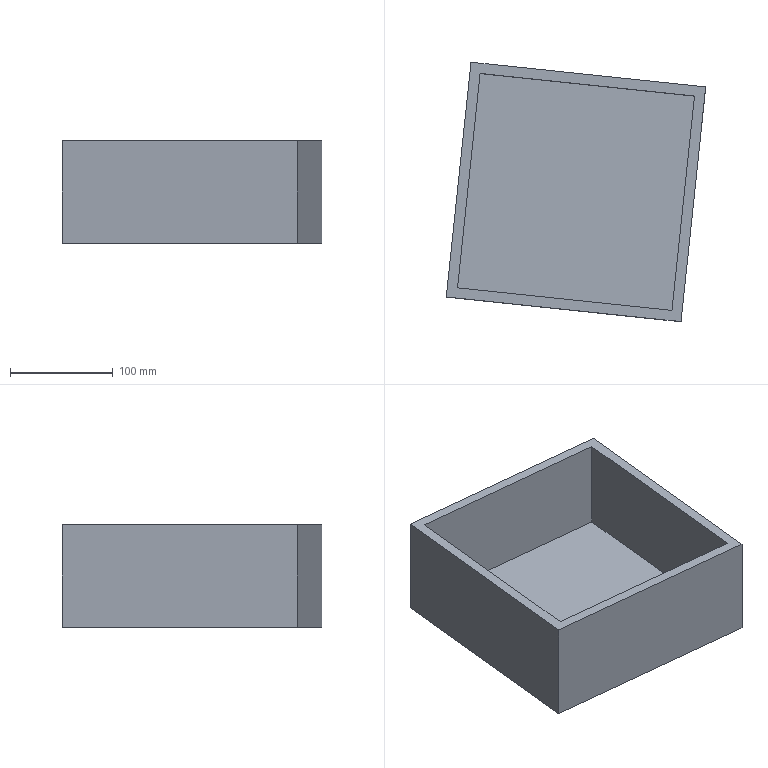Component | NX | SQUARE_BOX | 1 solid | 11 faces | box 252.78 x 252.78 x 100 mm | volume 1321000 mm3 | plane 11
STEP:
#1=CARTESIAN_POINT('',(0.,0.,0.));
#2=DIRECTION('',(0.,0.,1.));
#3=DIRECTION('',(1.,0.,0.));
#4=AXIS2_PLACEMENT_3D('',#1,#2,#3);
#5=CARTESIAN_POINT('',(-42.53,33.666,104.));
#6=VERTEX_POINT('',#5);
#7=CARTESIAN_POINT('',(-66.572,-195.074,104.));
#8=VERTEX_POINT('',#7);
#9=CARTESIAN_POINT('',(-54.551,-80.704,104.));
#10=DIRECTION('',(-0.1045,-0.9945,0.));
#11=VECTOR('',#10,1.);
#12=LINE('',#9,#11);
#13=CARTESIAN_POINT('',(-168.921,-68.683,104.));
#14=DIRECTION('',(0.,0.,1.));
#15=DIRECTION('',(0.1045,0.9945,0.));
#16=AXIS2_PLACEMENT_3D('',#13,#14,#15);
#17=PLANE('',#16);
#18=CARTESIAN_POINT('',(0.,-115.));
#19=DIRECTION('',(-1.,0.));
#20=VECTOR('',#19,1.);
#21=LINE('',#18,#20);
#22=(GEOMETRIC_REPRESENTATION_CONTEXT(2)PARAMETRIC_REPRESENTATION_CONTEXT()REPRESENTATION_CONTEXT('',''));
#23=DEFINITIONAL_REPRESENTATION('',(#21),#22);
#24=PCURVE('',#17,#23);
#25=CARTESIAN_POINT('',(-54.551,-80.704,4.));
#26=DIRECTION('',(0.9945,-0.1045,0.));
#27=DIRECTION('',(0.,0.,-1.));
#28=AXIS2_PLACEMENT_3D('',#25,#26,#27);
#29=PLANE('',#28);
#30=CARTESIAN_POINT('',(-100.,0.));
#31=DIRECTION('',(0.,-1.));
#32=VECTOR('',#31,1.);
#33=LINE('',#30,#32);
#34=(GEOMETRIC_REPRESENTATION_CONTEXT(2)PARAMETRIC_REPRESENTATION_CONTEXT()REPRESENTATION_CONTEXT('',''));
#35=DEFINITIONAL_REPRESENTATION('',(#33),#34);
#36=PCURVE('',#29,#35);
#37=SURFACE_CURVE('',#12,(#24,#36),.PCURVE_S1.);
#38=EDGE_CURVE('',#6,#8,#37,.T.);
#39=ORIENTED_EDGE('',*,*,#38,.F.);
#40=CARTESIAN_POINT('',(-271.27,57.707,104.));
#41=VERTEX_POINT('',#40);
#42=CARTESIAN_POINT('',(-156.9,45.687,104.));
#43=DIRECTION('',(0.9945,-0.1045,0.));
#44=VECTOR('',#43,1.);
#45=LINE('',#42,#44);
#46=CARTESIAN_POINT('',(115.,0.));
#47=DIRECTION('',(0.,-1.));
#48=VECTOR('',#47,1.);
#49=LINE('',#46,#48);
#50=(GEOMETRIC_REPRESENTATION_CONTEXT(2)PARAMETRIC_REPRESENTATION_CONTEXT()REPRESENTATION_CONTEXT('',''));
#51=DEFINITIONAL_REPRESENTATION('',(#49),#50);
#52=PCURVE('',#17,#51);
#53=CARTESIAN_POINT('',(-156.9,45.687,4.));
#54=DIRECTION('',(0.1045,0.9945,0.));
#55=DIRECTION('',(0.,0.,-1.));
#56=AXIS2_PLACEMENT_3D('',#53,#54,#55);
#57=PLANE('',#56);
#58=CARTESIAN_POINT('',(-100.,0.));
#59=DIRECTION('',(0.,-1.));
#60=VECTOR('',#59,1.);
#61=LINE('',#58,#60);
#62=(GEOMETRIC_REPRESENTATION_CONTEXT(2)PARAMETRIC_REPRESENTATION_CONTEXT()REPRESENTATION_CONTEXT('',''));
#63=DEFINITIONAL_REPRESENTATION('',(#61),#62);
#64=PCURVE('',#57,#63);
#65=SURFACE_CURVE('',#45,(#52,#64),.PCURVE_S1.);
#66=EDGE_CURVE('',#41,#6,#65,.T.);
#67=ORIENTED_EDGE('',*,*,#66,.F.);
#68=CARTESIAN_POINT('',(-295.312,-171.033,104.));
#69=VERTEX_POINT('',#68);
#70=CARTESIAN_POINT('',(-283.291,-56.663,104.));
#71=DIRECTION('',(0.1045,0.9945,0.));
#72=VECTOR('',#71,1.);
#73=LINE('',#70,#72);
#74=CARTESIAN_POINT('',(0.,115.));
#75=DIRECTION('',(1.,0.));
#76=VECTOR('',#75,1.);
#77=LINE('',#74,#76);
#78=(GEOMETRIC_REPRESENTATION_CONTEXT(2)PARAMETRIC_REPRESENTATION_CONTEXT()REPRESENTATION_CONTEXT('',''));
#79=DEFINITIONAL_REPRESENTATION('',(#77),#78);
#80=PCURVE('',#17,#79);
#81=CARTESIAN_POINT('',(-283.291,-56.663,4.));
#82=DIRECTION('',(-0.9945,0.1045,0.));
#83=DIRECTION('',(0.,0.,1.));
#84=AXIS2_PLACEMENT_3D('',#81,#82,#83);
#85=PLANE('',#84);
#86=CARTESIAN_POINT('',(100.,0.));
#87=DIRECTION('',(0.,1.));
#88=VECTOR('',#87,1.);
#89=LINE('',#86,#88);
#90=(GEOMETRIC_REPRESENTATION_CONTEXT(2)PARAMETRIC_REPRESENTATION_CONTEXT()REPRESENTATION_CONTEXT('',''));
#91=DEFINITIONAL_REPRESENTATION('',(#89),#90);
#92=PCURVE('',#85,#91);
#93=SURFACE_CURVE('',#73,(#80,#92),.PCURVE_S1.);
#94=EDGE_CURVE('',#69,#41,#93,.T.);
#95=ORIENTED_EDGE('',*,*,#94,.F.);
#96=CARTESIAN_POINT('',(-180.942,-183.053,104.));
#97=DIRECTION('',(-0.9945,0.1045,0.));
#98=VECTOR('',#97,1.);
#99=LINE('',#96,#98);
#100=CARTESIAN_POINT('',(-115.,-0.));
#101=DIRECTION('',(0.,1.));
#102=VECTOR('',#101,1.);
#103=LINE('',#100,#102);
#104=(GEOMETRIC_REPRESENTATION_CONTEXT(2)PARAMETRIC_REPRESENTATION_CONTEXT()REPRESENTATION_CONTEXT('',''));
#105=DEFINITIONAL_REPRESENTATION('',(#103),#104);
#106=PCURVE('',#17,#105);
#107=CARTESIAN_POINT('',(-180.942,-183.053,4.));
#108=DIRECTION('',(-0.1045,-0.9945,0.));
#109=DIRECTION('',(0.,0.,1.));
#110=AXIS2_PLACEMENT_3D('',#107,#108,#109);
#111=PLANE('',#110);
#112=CARTESIAN_POINT('',(100.,0.));
#113=DIRECTION('',(0.,1.));
#114=VECTOR('',#113,1.);
#115=LINE('',#112,#114);
#116=(GEOMETRIC_REPRESENTATION_CONTEXT(2)PARAMETRIC_REPRESENTATION_CONTEXT()REPRESENTATION_CONTEXT('',''));
#117=DEFINITIONAL_REPRESENTATION('',(#115),#116);
#118=PCURVE('',#111,#117);
#119=SURFACE_CURVE('',#99,(#106,#118),.PCURVE_S1.);
#120=EDGE_CURVE('',#8,#69,#119,.T.);
#121=ORIENTED_EDGE('',*,*,#120,.F.);
#122=EDGE_LOOP('',(#39,#67,#95,#121));
#123=FACE_BOUND('',#122,.T.);
#124=CARTESIAN_POINT('',(-262.37,46.717,104.));
#125=VERTEX_POINT('',#124);
#126=CARTESIAN_POINT('',(-53.521,24.766,104.));
#127=VERTEX_POINT('',#126);
#128=CARTESIAN_POINT('',(-157.946,35.741,104.));
#129=DIRECTION('',(0.9945,-0.1045,0.));
#130=VECTOR('',#129,1.);
#131=LINE('',#128,#130);
#132=CARTESIAN_POINT('',(105.,-0.));
#133=DIRECTION('',(0.,-1.));
#134=VECTOR('',#133,1.);
#135=LINE('',#132,#134);
#136=(GEOMETRIC_REPRESENTATION_CONTEXT(2)PARAMETRIC_REPRESENTATION_CONTEXT()REPRESENTATION_CONTEXT('',''));
#137=DEFINITIONAL_REPRESENTATION('',(#135),#136);
#138=PCURVE('',#17,#137);
#139=CARTESIAN_POINT('',(-157.946,35.741,4.));
#140=DIRECTION('',(0.1045,0.9945,0.));
#141=DIRECTION('',(0.,0.,-1.));
#142=AXIS2_PLACEMENT_3D('',#139,#140,#141);
#143=PLANE('',#142);
#144=CARTESIAN_POINT('',(-100.,0.));
#145=DIRECTION('',(0.,-1.));
#146=VECTOR('',#145,1.);
#147=LINE('',#144,#146);
#148=(GEOMETRIC_REPRESENTATION_CONTEXT(2)PARAMETRIC_REPRESENTATION_CONTEXT()REPRESENTATION_CONTEXT('',''));
#149=DEFINITIONAL_REPRESENTATION('',(#147),#148);
#150=PCURVE('',#143,#149);
#151=SURFACE_CURVE('',#131,(#138,#150),.PCURVE_S1.);
#152=EDGE_CURVE('',#125,#127,#151,.T.);
#153=ORIENTED_EDGE('',*,*,#152,.T.);
#154=CARTESIAN_POINT('',(-75.472,-184.084,104.));
#155=VERTEX_POINT('',#154);
#156=CARTESIAN_POINT('',(-64.496,-79.659,104.));
#157=DIRECTION('',(-0.1045,-0.9945,0.));
#158=VECTOR('',#157,1.);
#159=LINE('',#156,#158);
#160=CARTESIAN_POINT('',(-0.,-105.));
#161=DIRECTION('',(-1.,0.));
#162=VECTOR('',#161,1.);
#163=LINE('',#160,#162);
#164=(GEOMETRIC_REPRESENTATION_CONTEXT(2)PARAMETRIC_REPRESENTATION_CONTEXT()REPRESENTATION_CONTEXT('',''));
#165=DEFINITIONAL_REPRESENTATION('',(#163),#164);
#166=PCURVE('',#17,#165);
#167=CARTESIAN_POINT('',(-64.496,-79.659,4.));
#168=DIRECTION('',(0.9945,-0.1045,0.));
#169=DIRECTION('',(0.,0.,-1.));
#170=AXIS2_PLACEMENT_3D('',#167,#168,#169);
#171=PLANE('',#170);
#172=CARTESIAN_POINT('',(-100.,0.));
#173=DIRECTION('',(0.,-1.));
#174=VECTOR('',#173,1.);
#175=LINE('',#172,#174);
#176=(GEOMETRIC_REPRESENTATION_CONTEXT(2)PARAMETRIC_REPRESENTATION_CONTEXT()REPRESENTATION_CONTEXT('',''));
#177=DEFINITIONAL_REPRESENTATION('',(#175),#176);
#178=PCURVE('',#171,#177);
#179=SURFACE_CURVE('',#159,(#166,#178),.PCURVE_S1.);
#180=EDGE_CURVE('',#127,#155,#179,.T.);
#181=ORIENTED_EDGE('',*,*,#180,.T.);
#182=CARTESIAN_POINT('',(-284.321,-162.133,104.));
#183=VERTEX_POINT('',#182);
#184=CARTESIAN_POINT('',(-179.897,-173.108,104.));
#185=DIRECTION('',(-0.9945,0.1045,0.));
#186=VECTOR('',#185,1.);
#187=LINE('',#184,#186);
#188=CARTESIAN_POINT('',(-105.,-0.));
#189=DIRECTION('',(0.,1.));
#190=VECTOR('',#189,1.);
#191=LINE('',#188,#190);
#192=(GEOMETRIC_REPRESENTATION_CONTEXT(2)PARAMETRIC_REPRESENTATION_CONTEXT()REPRESENTATION_CONTEXT('',''));
#193=DEFINITIONAL_REPRESENTATION('',(#191),#192);
#194=PCURVE('',#17,#193);
#195=CARTESIAN_POINT('',(-179.897,-173.108,4.));
#196=DIRECTION('',(-0.1045,-0.9945,0.));
#197=DIRECTION('',(0.,0.,1.));
#198=AXIS2_PLACEMENT_3D('',#195,#196,#197);
#199=PLANE('',#198);
#200=CARTESIAN_POINT('',(100.,0.));
#201=DIRECTION('',(0.,1.));
#202=VECTOR('',#201,1.);
#203=LINE('',#200,#202);
#204=(GEOMETRIC_REPRESENTATION_CONTEXT(2)PARAMETRIC_REPRESENTATION_CONTEXT()REPRESENTATION_CONTEXT('',''));
#205=DEFINITIONAL_REPRESENTATION('',(#203),#204);
#206=PCURVE('',#199,#205);
#207=SURFACE_CURVE('',#187,(#194,#206),.PCURVE_S1.);
#208=EDGE_CURVE('',#155,#183,#207,.T.);
#209=ORIENTED_EDGE('',*,*,#208,.T.);
#210=CARTESIAN_POINT('',(-273.346,-57.708,104.));
#211=DIRECTION('',(0.1045,0.9945,0.));
#212=VECTOR('',#211,1.);
#213=LINE('',#210,#212);
#214=CARTESIAN_POINT('',(0.,105.));
#215=DIRECTION('',(1.,0.));
#216=VECTOR('',#215,1.);
#217=LINE('',#214,#216);
#218=(GEOMETRIC_REPRESENTATION_CONTEXT(2)PARAMETRIC_REPRESENTATION_CONTEXT()REPRESENTATION_CONTEXT('',''));
#219=DEFINITIONAL_REPRESENTATION('',(#217),#218);
#220=PCURVE('',#17,#219);
#221=CARTESIAN_POINT('',(-273.346,-57.708,4.));
#222=DIRECTION('',(-0.9945,0.1045,0.));
#223=DIRECTION('',(0.,0.,1.));
#224=AXIS2_PLACEMENT_3D('',#221,#222,#223);
#225=PLANE('',#224);
#226=CARTESIAN_POINT('',(100.,0.));
#227=DIRECTION('',(0.,1.));
#228=VECTOR('',#227,1.);
#229=LINE('',#226,#228);
#230=(GEOMETRIC_REPRESENTATION_CONTEXT(2)PARAMETRIC_REPRESENTATION_CONTEXT()REPRESENTATION_CONTEXT('',''));
#231=DEFINITIONAL_REPRESENTATION('',(#229),#230);
#232=PCURVE('',#225,#231);
#233=SURFACE_CURVE('',#213,(#220,#232),.PCURVE_S1.);
#234=EDGE_CURVE('',#183,#125,#233,.T.);
#235=ORIENTED_EDGE('',*,*,#234,.T.);
#236=EDGE_LOOP('',(#153,#181,#209,#235));
#237=FACE_BOUND('',#236,.T.);
#238=ADVANCED_FACE('',(#123,#237),#17,.T.);
#239=CARTESIAN_POINT('',(-42.53,33.666,4.));
#240=VERTEX_POINT('',#239);
#241=CARTESIAN_POINT('',(-42.53,33.666,4.));
#242=DIRECTION('',(0.,0.,1.));
#243=VECTOR('',#242,1.);
#244=LINE('',#241,#243);
#245=CARTESIAN_POINT('',(0.,115.));
#246=DIRECTION('',(-1.,0.));
#247=VECTOR('',#246,1.);
#248=LINE('',#245,#247);
#249=(GEOMETRIC_REPRESENTATION_CONTEXT(2)PARAMETRIC_REPRESENTATION_CONTEXT()REPRESENTATION_CONTEXT('',''));
#250=DEFINITIONAL_REPRESENTATION('',(#248),#249);
#251=PCURVE('',#29,#250);
#252=CARTESIAN_POINT('',(0.,-115.));
#253=DIRECTION('',(-1.,0.));
#254=VECTOR('',#253,1.);
#255=LINE('',#252,#254);
#256=(GEOMETRIC_REPRESENTATION_CONTEXT(2)PARAMETRIC_REPRESENTATION_CONTEXT()REPRESENTATION_CONTEXT('',''));
#257=DEFINITIONAL_REPRESENTATION('',(#255),#256);
#258=PCURVE('',#57,#257);
#259=SURFACE_CURVE('',#244,(#251,#258),.PCURVE_S1.);
#260=EDGE_CURVE('',#240,#6,#259,.T.);
#261=ORIENTED_EDGE('',*,*,#260,.T.);
#262=ORIENTED_EDGE('',*,*,#38,.T.);
#263=CARTESIAN_POINT('',(-66.572,-195.074,4.));
#264=VERTEX_POINT('',#263);
#265=CARTESIAN_POINT('',(-66.572,-195.074,4.));
#266=DIRECTION('',(0.,0.,1.));
#267=VECTOR('',#266,1.);
#268=LINE('',#265,#267);
#269=CARTESIAN_POINT('',(0.,-115.));
#270=DIRECTION('',(-1.,0.));
#271=VECTOR('',#270,1.);
#272=LINE('',#269,#271);
#273=(GEOMETRIC_REPRESENTATION_CONTEXT(2)PARAMETRIC_REPRESENTATION_CONTEXT()REPRESENTATION_CONTEXT('',''));
#274=DEFINITIONAL_REPRESENTATION('',(#272),#273);
#275=PCURVE('',#29,#274);
#276=CARTESIAN_POINT('',(0.,-115.));
#277=DIRECTION('',(1.,0.));
#278=VECTOR('',#277,1.);
#279=LINE('',#276,#278);
#280=(GEOMETRIC_REPRESENTATION_CONTEXT(2)PARAMETRIC_REPRESENTATION_CONTEXT()REPRESENTATION_CONTEXT('',''));
#281=DEFINITIONAL_REPRESENTATION('',(#279),#280);
#282=PCURVE('',#111,#281);
#283=SURFACE_CURVE('',#268,(#275,#282),.PCURVE_S1.);
#284=EDGE_CURVE('',#264,#8,#283,.T.);
#285=ORIENTED_EDGE('',*,*,#284,.F.);
#286=CARTESIAN_POINT('',(-54.551,-80.704,4.));
#287=DIRECTION('',(0.1045,0.9945,0.));
#288=VECTOR('',#287,1.);
#289=LINE('',#286,#288);
#290=CARTESIAN_POINT('',(0.,0.));
#291=DIRECTION('',(0.,1.));
#292=VECTOR('',#291,1.);
#293=LINE('',#290,#292);
#294=(GEOMETRIC_REPRESENTATION_CONTEXT(2)PARAMETRIC_REPRESENTATION_CONTEXT()REPRESENTATION_CONTEXT('',''));
#295=DEFINITIONAL_REPRESENTATION('',(#293),#294);
#296=PCURVE('',#29,#295);
#297=CARTESIAN_POINT('',(-168.921,-68.683,4.));
#298=DIRECTION('',(0.,0.,-1.));
#299=DIRECTION('',(-0.1045,-0.9945,0.));
#300=AXIS2_PLACEMENT_3D('',#297,#298,#299);
#301=PLANE('',#300);
#302=CARTESIAN_POINT('',(-0.,-115.));
#303=DIRECTION('',(-1.,0.));
#304=VECTOR('',#303,1.);
#305=LINE('',#302,#304);
#306=(GEOMETRIC_REPRESENTATION_CONTEXT(2)PARAMETRIC_REPRESENTATION_CONTEXT()REPRESENTATION_CONTEXT('',''));
#307=DEFINITIONAL_REPRESENTATION('',(#305),#306);
#308=PCURVE('',#301,#307);
#309=SURFACE_CURVE('',#289,(#296,#308),.PCURVE_S1.);
#310=EDGE_CURVE('',#264,#240,#309,.T.);
#311=ORIENTED_EDGE('',*,*,#310,.T.);
#312=EDGE_LOOP('',(#261,#262,#285,#311));
#313=FACE_BOUND('',#312,.T.);
#314=ADVANCED_FACE('',(#313),#29,.T.);
#315=ORIENTED_EDGE('',*,*,#284,.T.);
#316=ORIENTED_EDGE('',*,*,#120,.T.);
#317=CARTESIAN_POINT('',(-295.312,-171.033,4.));
#318=VERTEX_POINT('',#317);
#319=CARTESIAN_POINT('',(-295.312,-171.033,4.));
#320=DIRECTION('',(0.,0.,1.));
#321=VECTOR('',#320,1.);
#322=LINE('',#319,#321);
#323=CARTESIAN_POINT('',(0.,115.));
#324=DIRECTION('',(1.,0.));
#325=VECTOR('',#324,1.);
#326=LINE('',#323,#325);
#327=(GEOMETRIC_REPRESENTATION_CONTEXT(2)PARAMETRIC_REPRESENTATION_CONTEXT()REPRESENTATION_CONTEXT('',''));
#328=DEFINITIONAL_REPRESENTATION('',(#326),#327);
#329=PCURVE('',#111,#328);
#330=CARTESIAN_POINT('',(0.,-115.));
#331=DIRECTION('',(1.,0.));
#332=VECTOR('',#331,1.);
#333=LINE('',#330,#332);
#334=(GEOMETRIC_REPRESENTATION_CONTEXT(2)PARAMETRIC_REPRESENTATION_CONTEXT()REPRESENTATION_CONTEXT('',''));
#335=DEFINITIONAL_REPRESENTATION('',(#333),#334);
#336=PCURVE('',#85,#335);
#337=SURFACE_CURVE('',#322,(#329,#336),.PCURVE_S1.);
#338=EDGE_CURVE('',#318,#69,#337,.T.);
#339=ORIENTED_EDGE('',*,*,#338,.F.);
#340=CARTESIAN_POINT('',(-180.942,-183.053,4.));
#341=DIRECTION('',(0.9945,-0.1045,0.));
#342=VECTOR('',#341,1.);
#343=LINE('',#340,#342);
#344=CARTESIAN_POINT('',(0.,0.));
#345=DIRECTION('',(0.,-1.));
#346=VECTOR('',#345,1.);
#347=LINE('',#344,#346);
#348=(GEOMETRIC_REPRESENTATION_CONTEXT(2)PARAMETRIC_REPRESENTATION_CONTEXT()REPRESENTATION_CONTEXT('',''));
#349=DEFINITIONAL_REPRESENTATION('',(#347),#348);
#350=PCURVE('',#111,#349);
#351=CARTESIAN_POINT('',(115.,-0.));
#352=DIRECTION('',(-0.,-1.));
#353=VECTOR('',#352,1.);
#354=LINE('',#351,#353);
#355=(GEOMETRIC_REPRESENTATION_CONTEXT(2)PARAMETRIC_REPRESENTATION_CONTEXT()REPRESENTATION_CONTEXT('',''));
#356=DEFINITIONAL_REPRESENTATION('',(#354),#355);
#357=PCURVE('',#301,#356);
#358=SURFACE_CURVE('',#343,(#350,#357),.PCURVE_S1.);
#359=EDGE_CURVE('',#318,#264,#358,.T.);
#360=ORIENTED_EDGE('',*,*,#359,.T.);
#361=EDGE_LOOP('',(#315,#316,#339,#360));
#362=FACE_BOUND('',#361,.T.);
#363=ADVANCED_FACE('',(#362),#111,.T.);
#364=ORIENTED_EDGE('',*,*,#338,.T.);
#365=ORIENTED_EDGE('',*,*,#94,.T.);
#366=CARTESIAN_POINT('',(-271.27,57.707,4.));
#367=VERTEX_POINT('',#366);
#368=CARTESIAN_POINT('',(-271.27,57.707,4.));
#369=DIRECTION('',(0.,0.,1.));
#370=VECTOR('',#369,1.);
#371=LINE('',#368,#370);
#372=CARTESIAN_POINT('',(0.,115.));
#373=DIRECTION('',(1.,0.));
#374=VECTOR('',#373,1.);
#375=LINE('',#372,#374);
#376=(GEOMETRIC_REPRESENTATION_CONTEXT(2)PARAMETRIC_REPRESENTATION_CONTEXT()REPRESENTATION_CONTEXT('',''));
#377=DEFINITIONAL_REPRESENTATION('',(#375),#376);
#378=PCURVE('',#85,#377);
#379=CARTESIAN_POINT('',(0.,115.));
#380=DIRECTION('',(-1.,0.));
#381=VECTOR('',#380,1.);
#382=LINE('',#379,#381);
#383=(GEOMETRIC_REPRESENTATION_CONTEXT(2)PARAMETRIC_REPRESENTATION_CONTEXT()REPRESENTATION_CONTEXT('',''));
#384=DEFINITIONAL_REPRESENTATION('',(#382),#383);
#385=PCURVE('',#57,#384);
#386=SURFACE_CURVE('',#371,(#378,#385),.PCURVE_S1.);
#387=EDGE_CURVE('',#367,#41,#386,.T.);
#388=ORIENTED_EDGE('',*,*,#387,.F.);
#389=CARTESIAN_POINT('',(-283.291,-56.663,4.));
#390=DIRECTION('',(-0.1045,-0.9945,0.));
#391=VECTOR('',#390,1.);
#392=LINE('',#389,#391);
#393=CARTESIAN_POINT('',(0.,0.));
#394=DIRECTION('',(0.,-1.));
#395=VECTOR('',#394,1.);
#396=LINE('',#393,#395);
#397=(GEOMETRIC_REPRESENTATION_CONTEXT(2)PARAMETRIC_REPRESENTATION_CONTEXT()REPRESENTATION_CONTEXT('',''));
#398=DEFINITIONAL_REPRESENTATION('',(#396),#397);
#399=PCURVE('',#85,#398);
#400=CARTESIAN_POINT('',(-0.,115.));
#401=DIRECTION('',(1.,-0.));
#402=VECTOR('',#401,1.);
#403=LINE('',#400,#402);
#404=(GEOMETRIC_REPRESENTATION_CONTEXT(2)PARAMETRIC_REPRESENTATION_CONTEXT()REPRESENTATION_CONTEXT('',''));
#405=DEFINITIONAL_REPRESENTATION('',(#403),#404);
#406=PCURVE('',#301,#405);
#407=SURFACE_CURVE('',#392,(#399,#406),.PCURVE_S1.);
#408=EDGE_CURVE('',#367,#318,#407,.T.);
#409=ORIENTED_EDGE('',*,*,#408,.T.);
#410=EDGE_LOOP('',(#364,#365,#388,#409));
#411=FACE_BOUND('',#410,.T.);
#412=ADVANCED_FACE('',(#411),#85,.T.);
#413=CARTESIAN_POINT('',(-156.9,45.687,4.));
#414=DIRECTION('',(-0.9945,0.1045,0.));
#415=VECTOR('',#414,1.);
#416=LINE('',#413,#415);
#417=CARTESIAN_POINT('',(-115.,0.));
#418=DIRECTION('',(0.,1.));
#419=VECTOR('',#418,1.);
#420=LINE('',#417,#419);
#421=(GEOMETRIC_REPRESENTATION_CONTEXT(2)PARAMETRIC_REPRESENTATION_CONTEXT()REPRESENTATION_CONTEXT('',''));
#422=DEFINITIONAL_REPRESENTATION('',(#420),#421);
#423=PCURVE('',#301,#422);
#424=CARTESIAN_POINT('',(0.,0.));
#425=DIRECTION('',(0.,1.));
#426=VECTOR('',#425,1.);
#427=LINE('',#424,#426);
#428=(GEOMETRIC_REPRESENTATION_CONTEXT(2)PARAMETRIC_REPRESENTATION_CONTEXT()REPRESENTATION_CONTEXT('',''));
#429=DEFINITIONAL_REPRESENTATION('',(#427),#428);
#430=PCURVE('',#57,#429);
#431=SURFACE_CURVE('',#416,(#423,#430),.PCURVE_S1.);
#432=EDGE_CURVE('',#240,#367,#431,.T.);
#433=ORIENTED_EDGE('',*,*,#432,.F.);
#434=ORIENTED_EDGE('',*,*,#310,.F.);
#435=ORIENTED_EDGE('',*,*,#359,.F.);
#436=ORIENTED_EDGE('',*,*,#408,.F.);
#437=EDGE_LOOP('',(#433,#434,#435,#436));
#438=FACE_BOUND('',#437,.T.);
#439=ADVANCED_FACE('',(#438),#301,.T.);
#440=ORIENTED_EDGE('',*,*,#432,.T.);
#441=ORIENTED_EDGE('',*,*,#387,.T.);
#442=ORIENTED_EDGE('',*,*,#66,.T.);
#443=ORIENTED_EDGE('',*,*,#260,.F.);
#444=EDGE_LOOP('',(#440,#441,#442,#443));
#445=FACE_BOUND('',#444,.T.);
#446=ADVANCED_FACE('',(#445),#57,.T.);
#447=CARTESIAN_POINT('',(-53.521,24.766,14.));
#448=VERTEX_POINT('',#447);
#449=CARTESIAN_POINT('',(-53.521,24.766,4.));
#450=DIRECTION('',(0.,0.,1.));
#451=VECTOR('',#450,1.);
#452=LINE('',#449,#451);
#453=CARTESIAN_POINT('',(0.,105.));
#454=DIRECTION('',(-1.,0.));
#455=VECTOR('',#454,1.);
#456=LINE('',#453,#455);
#457=(GEOMETRIC_REPRESENTATION_CONTEXT(2)PARAMETRIC_REPRESENTATION_CONTEXT()REPRESENTATION_CONTEXT('',''));
#458=DEFINITIONAL_REPRESENTATION('',(#456),#457);
#459=PCURVE('',#171,#458);
#460=CARTESIAN_POINT('',(0.,-105.));
#461=DIRECTION('',(-1.,0.));
#462=VECTOR('',#461,1.);
#463=LINE('',#460,#462);
#464=(GEOMETRIC_REPRESENTATION_CONTEXT(2)PARAMETRIC_REPRESENTATION_CONTEXT()REPRESENTATION_CONTEXT('',''));
#465=DEFINITIONAL_REPRESENTATION('',(#463),#464);
#466=PCURVE('',#143,#465);
#467=SURFACE_CURVE('',#452,(#459,#466),.PCURVE_S1.);
#468=EDGE_CURVE('',#448,#127,#467,.T.);
#469=ORIENTED_EDGE('',*,*,#468,.F.);
#470=CARTESIAN_POINT('',(-75.472,-184.084,14.));
#471=VERTEX_POINT('',#470);
#472=CARTESIAN_POINT('',(-64.496,-79.659,14.));
#473=DIRECTION('',(0.1045,0.9945,0.));
#474=VECTOR('',#473,1.);
#475=LINE('',#472,#474);
#476=CARTESIAN_POINT('',(-10.,0.));
#477=DIRECTION('',(0.,1.));
#478=VECTOR('',#477,1.);
#479=LINE('',#476,#478);
#480=(GEOMETRIC_REPRESENTATION_CONTEXT(2)PARAMETRIC_REPRESENTATION_CONTEXT()REPRESENTATION_CONTEXT('',''));
#481=DEFINITIONAL_REPRESENTATION('',(#479),#480);
#482=PCURVE('',#171,#481);
#483=CARTESIAN_POINT('',(-168.921,-68.683,14.));
#484=DIRECTION('',(0.,0.,-1.));
#485=DIRECTION('',(-0.1045,-0.9945,0.));
#486=AXIS2_PLACEMENT_3D('',#483,#484,#485);
#487=PLANE('',#486);
#488=CARTESIAN_POINT('',(0.,-105.));
#489=DIRECTION('',(-1.,0.));
#490=VECTOR('',#489,1.);
#491=LINE('',#488,#490);
#492=(GEOMETRIC_REPRESENTATION_CONTEXT(2)PARAMETRIC_REPRESENTATION_CONTEXT()REPRESENTATION_CONTEXT('',''));
#493=DEFINITIONAL_REPRESENTATION('',(#491),#492);
#494=PCURVE('',#487,#493);
#495=SURFACE_CURVE('',#475,(#482,#494),.PCURVE_S1.);
#496=EDGE_CURVE('',#471,#448,#495,.T.);
#497=ORIENTED_EDGE('',*,*,#496,.F.);
#498=CARTESIAN_POINT('',(-75.472,-184.084,4.));
#499=DIRECTION('',(0.,0.,1.));
#500=VECTOR('',#499,1.);
#501=LINE('',#498,#500);
#502=CARTESIAN_POINT('',(0.,-105.));
#503=DIRECTION('',(-1.,0.));
#504=VECTOR('',#503,1.);
#505=LINE('',#502,#504);
#506=(GEOMETRIC_REPRESENTATION_CONTEXT(2)PARAMETRIC_REPRESENTATION_CONTEXT()REPRESENTATION_CONTEXT('',''));
#507=DEFINITIONAL_REPRESENTATION('',(#505),#506);
#508=PCURVE('',#171,#507);
#509=CARTESIAN_POINT('',(0.,-105.));
#510=DIRECTION('',(1.,0.));
#511=VECTOR('',#510,1.);
#512=LINE('',#509,#511);
#513=(GEOMETRIC_REPRESENTATION_CONTEXT(2)PARAMETRIC_REPRESENTATION_CONTEXT()REPRESENTATION_CONTEXT('',''));
#514=DEFINITIONAL_REPRESENTATION('',(#512),#513);
#515=PCURVE('',#199,#514);
#516=SURFACE_CURVE('',#501,(#508,#515),.PCURVE_S1.);
#517=EDGE_CURVE('',#471,#155,#516,.T.);
#518=ORIENTED_EDGE('',*,*,#517,.T.);
#519=ORIENTED_EDGE('',*,*,#180,.F.);
#520=EDGE_LOOP('',(#469,#497,#518,#519));
#521=FACE_BOUND('',#520,.T.);
#522=ADVANCED_FACE('',(#521),#171,.F.);
#523=ORIENTED_EDGE('',*,*,#517,.F.);
#524=CARTESIAN_POINT('',(-284.321,-162.133,14.));
#525=VERTEX_POINT('',#524);
#526=CARTESIAN_POINT('',(-179.897,-173.108,14.));
#527=DIRECTION('',(0.9945,-0.1045,0.));
#528=VECTOR('',#527,1.);
#529=LINE('',#526,#528);
#530=CARTESIAN_POINT('',(10.,0.));
#531=DIRECTION('',(0.,-1.));
#532=VECTOR('',#531,1.);
#533=LINE('',#530,#532);
#534=(GEOMETRIC_REPRESENTATION_CONTEXT(2)PARAMETRIC_REPRESENTATION_CONTEXT()REPRESENTATION_CONTEXT('',''));
#535=DEFINITIONAL_REPRESENTATION('',(#533),#534);
#536=PCURVE('',#199,#535);
#537=CARTESIAN_POINT('',(105.,-0.));
#538=DIRECTION('',(-0.,-1.));
#539=VECTOR('',#538,1.);
#540=LINE('',#537,#539);
#541=(GEOMETRIC_REPRESENTATION_CONTEXT(2)PARAMETRIC_REPRESENTATION_CONTEXT()REPRESENTATION_CONTEXT('',''));
#542=DEFINITIONAL_REPRESENTATION('',(#540),#541);
#543=PCURVE('',#487,#542);
#544=SURFACE_CURVE('',#529,(#536,#543),.PCURVE_S1.);
#545=EDGE_CURVE('',#525,#471,#544,.T.);
#546=ORIENTED_EDGE('',*,*,#545,.F.);
#547=CARTESIAN_POINT('',(-284.321,-162.133,4.));
#548=DIRECTION('',(0.,0.,1.));
#549=VECTOR('',#548,1.);
#550=LINE('',#547,#549);
#551=CARTESIAN_POINT('',(0.,105.));
#552=DIRECTION('',(1.,0.));
#553=VECTOR('',#552,1.);
#554=LINE('',#551,#553);
#555=(GEOMETRIC_REPRESENTATION_CONTEXT(2)PARAMETRIC_REPRESENTATION_CONTEXT()REPRESENTATION_CONTEXT('',''));
#556=DEFINITIONAL_REPRESENTATION('',(#554),#555);
#557=PCURVE('',#199,#556);
#558=CARTESIAN_POINT('',(0.,-105.));
#559=DIRECTION('',(1.,0.));
#560=VECTOR('',#559,1.);
#561=LINE('',#558,#560);
#562=(GEOMETRIC_REPRESENTATION_CONTEXT(2)PARAMETRIC_REPRESENTATION_CONTEXT()REPRESENTATION_CONTEXT('',''));
#563=DEFINITIONAL_REPRESENTATION('',(#561),#562);
#564=PCURVE('',#225,#563);
#565=SURFACE_CURVE('',#550,(#557,#564),.PCURVE_S1.);
#566=EDGE_CURVE('',#525,#183,#565,.T.);
#567=ORIENTED_EDGE('',*,*,#566,.T.);
#568=ORIENTED_EDGE('',*,*,#208,.F.);
#569=EDGE_LOOP('',(#523,#546,#567,#568));
#570=FACE_BOUND('',#569,.T.);
#571=ADVANCED_FACE('',(#570),#199,.F.);
#572=ORIENTED_EDGE('',*,*,#566,.F.);
#573=CARTESIAN_POINT('',(-262.37,46.717,14.));
#574=VERTEX_POINT('',#573);
#575=CARTESIAN_POINT('',(-273.346,-57.708,14.));
#576=DIRECTION('',(-0.1045,-0.9945,0.));
#577=VECTOR('',#576,1.);
#578=LINE('',#575,#577);
#579=CARTESIAN_POINT('',(10.,0.));
#580=DIRECTION('',(0.,-1.));
#581=VECTOR('',#580,1.);
#582=LINE('',#579,#581);
#583=(GEOMETRIC_REPRESENTATION_CONTEXT(2)PARAMETRIC_REPRESENTATION_CONTEXT()REPRESENTATION_CONTEXT('',''));
#584=DEFINITIONAL_REPRESENTATION('',(#582),#583);
#585=PCURVE('',#225,#584);
#586=CARTESIAN_POINT('',(-0.,105.));
#587=DIRECTION('',(1.,-0.));
#588=VECTOR('',#587,1.);
#589=LINE('',#586,#588);
#590=(GEOMETRIC_REPRESENTATION_CONTEXT(2)PARAMETRIC_REPRESENTATION_CONTEXT()REPRESENTATION_CONTEXT('',''));
#591=DEFINITIONAL_REPRESENTATION('',(#589),#590);
#592=PCURVE('',#487,#591);
#593=SURFACE_CURVE('',#578,(#585,#592),.PCURVE_S1.);
#594=EDGE_CURVE('',#574,#525,#593,.T.);
#595=ORIENTED_EDGE('',*,*,#594,.F.);
#596=CARTESIAN_POINT('',(-262.37,46.717,4.));
#597=DIRECTION('',(0.,0.,1.));
#598=VECTOR('',#597,1.);
#599=LINE('',#596,#598);
#600=CARTESIAN_POINT('',(0.,105.));
#601=DIRECTION('',(1.,0.));
#602=VECTOR('',#601,1.);
#603=LINE('',#600,#602);
#604=(GEOMETRIC_REPRESENTATION_CONTEXT(2)PARAMETRIC_REPRESENTATION_CONTEXT()REPRESENTATION_CONTEXT('',''));
#605=DEFINITIONAL_REPRESENTATION('',(#603),#604);
#606=PCURVE('',#225,#605);
#607=CARTESIAN_POINT('',(0.,105.));
#608=DIRECTION('',(-1.,0.));
#609=VECTOR('',#608,1.);
#610=LINE('',#607,#609);
#611=(GEOMETRIC_REPRESENTATION_CONTEXT(2)PARAMETRIC_REPRESENTATION_CONTEXT()REPRESENTATION_CONTEXT('',''));
#612=DEFINITIONAL_REPRESENTATION('',(#610),#611);
#613=PCURVE('',#143,#612);
#614=SURFACE_CURVE('',#599,(#606,#613),.PCURVE_S1.);
#615=EDGE_CURVE('',#574,#125,#614,.T.);
#616=ORIENTED_EDGE('',*,*,#615,.T.);
#617=ORIENTED_EDGE('',*,*,#234,.F.);
#618=EDGE_LOOP('',(#572,#595,#616,#617));
#619=FACE_BOUND('',#618,.T.);
#620=ADVANCED_FACE('',(#619),#225,.F.);
#621=CARTESIAN_POINT('',(-157.946,35.741,14.));
#622=DIRECTION('',(-0.9945,0.1045,0.));
#623=VECTOR('',#622,1.);
#624=LINE('',#621,#623);
#625=CARTESIAN_POINT('',(-105.,-0.));
#626=DIRECTION('',(0.,1.));
#627=VECTOR('',#626,1.);
#628=LINE('',#625,#627);
#629=(GEOMETRIC_REPRESENTATION_CONTEXT(2)PARAMETRIC_REPRESENTATION_CONTEXT()REPRESENTATION_CONTEXT('',''));
#630=DEFINITIONAL_REPRESENTATION('',(#628),#629);
#631=PCURVE('',#487,#630);
#632=CARTESIAN_POINT('',(-10.,0.));
#633=DIRECTION('',(0.,1.));
#634=VECTOR('',#633,1.);
#635=LINE('',#632,#634);
#636=(GEOMETRIC_REPRESENTATION_CONTEXT(2)PARAMETRIC_REPRESENTATION_CONTEXT()REPRESENTATION_CONTEXT('',''));
#637=DEFINITIONAL_REPRESENTATION('',(#635),#636);
#638=PCURVE('',#143,#637);
#639=SURFACE_CURVE('',#624,(#631,#638),.PCURVE_S1.);
#640=EDGE_CURVE('',#448,#574,#639,.T.);
#641=ORIENTED_EDGE('',*,*,#640,.T.);
#642=ORIENTED_EDGE('',*,*,#594,.T.);
#643=ORIENTED_EDGE('',*,*,#545,.T.);
#644=ORIENTED_EDGE('',*,*,#496,.T.);
#645=EDGE_LOOP('',(#641,#642,#643,#644));
#646=FACE_BOUND('',#645,.T.);
#647=ADVANCED_FACE('',(#646),#487,.F.);
#648=ORIENTED_EDGE('',*,*,#640,.F.);
#649=ORIENTED_EDGE('',*,*,#468,.T.);
#650=ORIENTED_EDGE('',*,*,#152,.F.);
#651=ORIENTED_EDGE('',*,*,#615,.F.);
#652=EDGE_LOOP('',(#648,#649,#650,#651));
#653=FACE_BOUND('',#652,.T.);
#654=ADVANCED_FACE('',(#653),#143,.F.);
#655=CLOSED_SHELL('',(#238,#314,#363,#412,#439,#446,#522,#571,#620,#647,#654));
#656=MANIFOLD_SOLID_BREP('',#655);
#657=(LENGTH_UNIT()NAMED_UNIT(*)SI_UNIT(.MILLI.,.METRE.));
#658=UNCERTAINTY_MEASURE_WITH_UNIT(LENGTH_MEASURE(0.0000001),#657,'','');
#659=(NAMED_UNIT(*)PLANE_ANGLE_UNIT()SI_UNIT($,.RADIAN.));
#660=(NAMED_UNIT(*)SI_UNIT($,.STERADIAN.)SOLID_ANGLE_UNIT());
#661=(GEOMETRIC_REPRESENTATION_CONTEXT(3)GLOBAL_UNCERTAINTY_ASSIGNED_CONTEXT((#658))GLOBAL_UNIT_ASSIGNED_CONTEXT((#657,#659,#660))REPRESENTATION_CONTEXT('',''));
#662=ADVANCED_BREP_SHAPE_REPRESENTATION('',(#4,#656),#661);